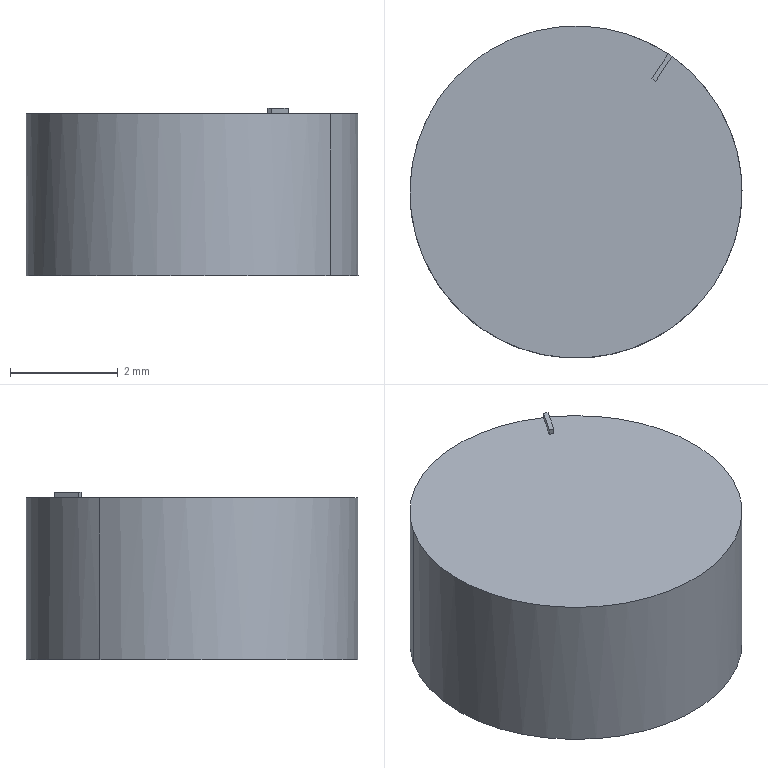Component | SolidWorks | Button-1 | 1 solid | 12 faces | box 6.16 x 6.16 x 3.1 mm | volume 88 mm3 | plane 8 | cylinder 4 | commonest cylinder face diameters 1 x2 6.16 x2
build123d program:
from build123d import *

# Parameters (mm, degrees)
SKETCH1_R           = 3.08
BOSS_EXTRUDE1_DEPTH = 3
SKETCH2_R           = 0.5
CUT_EXTRUDE1_DEPTH  = 2
SKETCH3_W           = 0.08765
SKETCH3_H           = 0.5469
BOSS_EXTRUDE2_DEPTH = 0.1


with BuildPart() as part:
    # Sketch1 → Boss-Extrude1 (new body)
    with BuildSketch(Plane.XY):
        Circle(SKETCH1_R)
    extrude(amount=BOSS_EXTRUDE1_DEPTH)

    # Sketch2 → Cut-Extrude1 (cut)
    with BuildSketch(Plane(origin=(0, 0, 0), x_dir=(-1, 0, 0), z_dir=(0, 0, -1))):
        Circle(SKETCH2_R)
    extrude(amount=-CUT_EXTRUDE1_DEPTH, mode=Mode.SUBTRACT)

    # Sketch3 → Boss-Extrude2 (add)
    with BuildSketch(Plane.XY.offset(3)):
        with Locations((0.04383, 2.807)):
            Rectangle(SKETCH3_W, SKETCH3_H)
    extrude(amount=BOSS_EXTRUDE2_DEPTH)


solid = part.part

# Placed as in the assembly
solid = solid.moved(Location((-92.68, 2.928, 277.152), (0.0002446, -0.0002387, -33.708)))
STEP:
#1=COLOUR_RGB('',0.7922,0.8196,0.9333);
#2=FILL_AREA_STYLE_COLOUR('',#1);
#3=FILL_AREA_STYLE('',(#2));
#4=SURFACE_STYLE_FILL_AREA(#3);
#5=SURFACE_SIDE_STYLE('',(#4));
#6=SURFACE_STYLE_USAGE(.BOTH.,#5);
#7=PRESENTATION_STYLE_ASSIGNMENT((#6));
#8=CARTESIAN_POINT('',(-3.632,0.1044,10.99));
#9=VERTEX_POINT('',#8);
#10=CARTESIAN_POINT('',(-3.665,0.1262,10.99));
#11=VERTEX_POINT('',#10);
#12=CARTESIAN_POINT('',(-3.649,0.1153,10.99));
#13=DIRECTION('',(0.,0.,-1.));
#14=DIRECTION('',(-0.8318,0.5551,0.));
#15=AXIS2_PLACEMENT_3D('',#12,#13,#14);
#16=CIRCLE('',#15,0.01969);
#17=EDGE_CURVE('',#9,#11,#16,.T.);
#18=ORIENTED_EDGE('',*,*,#17,.F.);
#19=CARTESIAN_POINT('',(-3.632,0.1044,10.911));
#20=VERTEX_POINT('',#19);
#21=CARTESIAN_POINT('',(-3.632,0.1044,10.99));
#22=DIRECTION('',(0.,0.,-1.));
#23=VECTOR('',#22,39.37);
#24=LINE('',#21,#23);
#25=EDGE_CURVE('',#9,#20,#24,.T.);
#26=ORIENTED_EDGE('',*,*,#25,.T.);
#27=CARTESIAN_POINT('',(-3.665,0.1262,10.911));
#28=VERTEX_POINT('',#27);
#29=CARTESIAN_POINT('',(-3.649,0.1153,10.911));
#30=DIRECTION('',(0.,0.,-1.));
#31=DIRECTION('',(-0.8318,0.5551,0.));
#32=AXIS2_PLACEMENT_3D('',#29,#30,#31);
#33=CIRCLE('',#32,0.01969);
#34=EDGE_CURVE('',#20,#28,#33,.T.);
#35=ORIENTED_EDGE('',*,*,#34,.T.);
#36=CARTESIAN_POINT('',(-3.665,0.1262,10.99));
#37=DIRECTION('',(0.,0.,-1.));
#38=VECTOR('',#37,39.37);
#39=LINE('',#36,#38);
#40=EDGE_CURVE('',#11,#28,#39,.T.);
#41=ORIENTED_EDGE('',*,*,#40,.F.);
#42=EDGE_LOOP('',(#18,#26,#35,#41));
#43=FACE_OUTER_BOUND('',#42,.T.);
#44=CARTESIAN_POINT('',(-3.649,0.1153,10.99));
#45=DIRECTION('',(0.,0.,-1.));
#46=DIRECTION('',(-0.8318,0.5551,0.));
#47=AXIS2_PLACEMENT_3D('',#44,#45,#46);
#48=CYLINDRICAL_SURFACE('',#47,0.01969);
#49=ADVANCED_FACE('',(#43),#48,.F.);
#50=CARTESIAN_POINT('',(-3.548,0.04799,11.03));
#51=VERTEX_POINT('',#50);
#52=CARTESIAN_POINT('',(-3.579,0.2142,11.03));
#53=VERTEX_POINT('',#52);
#54=CARTESIAN_POINT('',(-3.548,0.04799,11.03));
#55=CARTESIAN_POINT('',(-3.539,0.06111,11.03));
#56=CARTESIAN_POINT('',(-3.533,0.07541,11.03));
#57=CARTESIAN_POINT('',(-3.527,0.1063,11.03));
#58=CARTESIAN_POINT('',(-3.527,0.1218,11.03));
#59=CARTESIAN_POINT('',(-3.532,0.1528,11.03));
#60=CARTESIAN_POINT('',(-3.538,0.1673,11.03));
#61=CARTESIAN_POINT('',(-3.555,0.1938,11.03));
#62=CARTESIAN_POINT('',(-3.566,0.2051,11.03));
#63=CARTESIAN_POINT('',(-3.579,0.2142,11.03));
#64=B_SPLINE_CURVE_WITH_KNOTS('',3,(#54,#55,#56,#57,#58,#59,#60,#61,#62,#63),.UNSPECIFIED.,.F.,.F.,(4,2,2,2,4),(0.,0.06138,0.1228,0.1841,0.2455),.UNSPECIFIED.);
#65=EDGE_CURVE('',#51,#53,#64,.T.);
#66=ORIENTED_EDGE('',*,*,#65,.F.);
#67=CARTESIAN_POINT('',(-3.548,0.04799,10.911));
#68=VERTEX_POINT('',#67);
#69=CARTESIAN_POINT('',(-3.548,0.04799,11.03));
#70=DIRECTION('',(0.,0.,-1.));
#71=VECTOR('',#70,39.37);
#72=LINE('',#69,#71);
#73=EDGE_CURVE('',#51,#68,#72,.T.);
#74=ORIENTED_EDGE('',*,*,#73,.T.);
#75=CARTESIAN_POINT('',(-3.75,0.1826,10.911));
#76=VERTEX_POINT('',#75);
#77=CARTESIAN_POINT('',(-3.649,0.1153,10.911));
#78=DIRECTION('',(0.,0.,1.));
#79=DIRECTION('',(0.8318,-0.5551,0.));
#80=AXIS2_PLACEMENT_3D('',#77,#78,#79);
#81=CIRCLE('',#80,0.1213);
#82=EDGE_CURVE('',#68,#76,#81,.T.);
#83=ORIENTED_EDGE('',*,*,#82,.T.);
#84=CARTESIAN_POINT('',(-3.75,0.1826,11.03));
#85=VERTEX_POINT('',#84);
#86=CARTESIAN_POINT('',(-3.75,0.1826,11.03));
#87=DIRECTION('',(0.,0.,-1.));
#88=VECTOR('',#87,39.37);
#89=LINE('',#86,#88);
#90=EDGE_CURVE('',#85,#76,#89,.T.);
#91=ORIENTED_EDGE('',*,*,#90,.F.);
#92=CARTESIAN_POINT('',(-3.582,0.2162,11.03));
#93=VERTEX_POINT('',#92);
#94=CARTESIAN_POINT('',(-3.582,0.2162,11.03));
#95=CARTESIAN_POINT('',(-3.595,0.2251,11.03));
#96=CARTESIAN_POINT('',(-3.609,0.2311,11.03));
#97=CARTESIAN_POINT('',(-3.641,0.2374,11.03));
#98=CARTESIAN_POINT('',(-3.657,0.2373,11.03));
#99=CARTESIAN_POINT('',(-3.688,0.2311,11.03));
#100=CARTESIAN_POINT('',(-3.703,0.225,11.03));
#101=CARTESIAN_POINT('',(-3.73,0.2071,11.03));
#102=CARTESIAN_POINT('',(-3.741,0.196,11.03));
#103=CARTESIAN_POINT('',(-3.75,0.1826,11.03));
#104=B_SPLINE_CURVE_WITH_KNOTS('',3,(#94,#95,#96,#97,#98,#99,#100,#101,#102,#103),.UNSPECIFIED.,.F.,.F.,(4,2,2,2,4),(0.25,0.3125,0.375,0.4375,0.5),.UNSPECIFIED.);
#105=EDGE_CURVE('',#93,#85,#104,.T.);
#106=ORIENTED_EDGE('',*,*,#105,.F.);
#107=CARTESIAN_POINT('',(-3.579,0.2142,11.03));
#108=CARTESIAN_POINT('',(-3.58,0.2149,11.03));
#109=CARTESIAN_POINT('',(-3.581,0.2155,11.03));
#110=CARTESIAN_POINT('',(-3.582,0.2162,11.03));
#111=B_SPLINE_CURVE_WITH_KNOTS('',3,(#107,#108,#109,#110),.UNSPECIFIED.,.F.,.F.,(4,4),(0.,1.),.UNSPECIFIED.);
#112=EDGE_CURVE('',#53,#93,#111,.T.);
#113=ORIENTED_EDGE('',*,*,#112,.F.);
#114=EDGE_LOOP('',(#66,#74,#83,#91,#106,#113));
#115=FACE_OUTER_BOUND('',#114,.T.);
#116=CARTESIAN_POINT('',(-3.649,0.1153,11.03));
#117=DIRECTION('',(0.,0.,-1.));
#118=DIRECTION('',(-0.8318,0.5551,0.));
#119=AXIS2_PLACEMENT_3D('',#116,#117,#118);
#120=CYLINDRICAL_SURFACE('',#119,0.1213);
#121=ADVANCED_FACE('',(#115),#120,.T.);
#122=ORIENTED_EDGE('',*,*,#73,.F.);
#123=CARTESIAN_POINT('',(-3.75,0.1826,11.03));
#124=CARTESIAN_POINT('',(-3.759,0.1692,11.03));
#125=CARTESIAN_POINT('',(-3.765,0.1546,11.03));
#126=CARTESIAN_POINT('',(-3.771,0.1231,11.03));
#127=CARTESIAN_POINT('',(-3.771,0.1073,11.03));
#128=CARTESIAN_POINT('',(-3.765,0.07581,11.03));
#129=CARTESIAN_POINT('',(-3.759,0.06121,11.03));
#130=CARTESIAN_POINT('',(-3.741,0.03451,11.03));
#131=CARTESIAN_POINT('',(-3.729,0.02334,11.03));
#132=CARTESIAN_POINT('',(-3.703,0.005509,11.03));
#133=CARTESIAN_POINT('',(-3.688,-0.0005247,11.03));
#134=CARTESIAN_POINT('',(-3.657,-0.006779,11.03));
#135=CARTESIAN_POINT('',(-3.641,-0.006762,11.03));
#136=CARTESIAN_POINT('',(-3.609,-0.0004839,11.03));
#137=CARTESIAN_POINT('',(-3.595,0.005577,11.03));
#138=CARTESIAN_POINT('',(-3.568,0.02344,11.03));
#139=CARTESIAN_POINT('',(-3.557,0.0346,11.03));
#140=CARTESIAN_POINT('',(-3.548,0.04799,11.03));
#141=B_SPLINE_CURVE_WITH_KNOTS('',3,(#123,#124,#125,#126,#127,#128,#129,#130,#131,#132,#133,#134,#135,#136,#137,#138,#139,#140),.UNSPECIFIED.,.F.,.F.,(4,2,2,2,2,2,2,2,4),(0.5,0.5625,0.625,0.6875,0.75,0.8125,0.875,0.9375,1.),.UNSPECIFIED.);
#142=EDGE_CURVE('',#85,#51,#141,.T.);
#143=ORIENTED_EDGE('',*,*,#142,.F.);
#144=ORIENTED_EDGE('',*,*,#90,.T.);
#145=CARTESIAN_POINT('',(-3.649,0.1153,10.911));
#146=DIRECTION('',(0.,0.,1.));
#147=DIRECTION('',(0.8318,-0.5551,0.));
#148=AXIS2_PLACEMENT_3D('',#145,#146,#147);
#149=CIRCLE('',#148,0.1213);
#150=EDGE_CURVE('',#76,#68,#149,.T.);
#151=ORIENTED_EDGE('',*,*,#150,.T.);
#152=EDGE_LOOP('',(#122,#143,#144,#151));
#153=FACE_OUTER_BOUND('',#152,.T.);
#154=CARTESIAN_POINT('',(-3.649,0.1153,11.03));
#155=DIRECTION('',(0.,0.,-1.));
#156=DIRECTION('',(-0.8318,0.5551,0.));
#157=AXIS2_PLACEMENT_3D('',#154,#155,#156);
#158=CYLINDRICAL_SURFACE('',#157,0.1213);
#159=ADVANCED_FACE('',(#153),#158,.T.);
#160=CARTESIAN_POINT('',(-3.593,0.1982,11.03));
#161=VERTEX_POINT('',#160);
#162=CARTESIAN_POINT('',(-3.582,0.2162,11.03));
#163=DIRECTION('',(-0.5551,-0.8318,0.));
#164=VECTOR('',#163,39.37);
#165=LINE('',#162,#164);
#166=EDGE_CURVE('',#93,#161,#165,.T.);
#167=ORIENTED_EDGE('',*,*,#166,.F.);
#168=ORIENTED_EDGE('',*,*,#105,.T.);
#169=ORIENTED_EDGE('',*,*,#142,.T.);
#170=ORIENTED_EDGE('',*,*,#65,.T.);
#171=CARTESIAN_POINT('',(-3.591,0.1963,11.03));
#172=VERTEX_POINT('',#171);
#173=CARTESIAN_POINT('',(-3.579,0.2142,11.03));
#174=DIRECTION('',(0.5551,0.8318,0.));
#175=VECTOR('',#174,39.37);
#176=LINE('',#173,#175);
#177=EDGE_CURVE('',#172,#53,#176,.T.);
#178=ORIENTED_EDGE('',*,*,#177,.F.);
#179=CARTESIAN_POINT('',(-3.593,0.1982,11.03));
#180=DIRECTION('',(0.8318,-0.5551,0.));
#181=VECTOR('',#180,39.37);
#182=LINE('',#179,#181);
#183=EDGE_CURVE('',#161,#172,#182,.T.);
#184=ORIENTED_EDGE('',*,*,#183,.F.);
#185=EDGE_LOOP('',(#167,#168,#169,#170,#178,#184));
#186=FACE_OUTER_BOUND('',#185,.T.);
#187=CARTESIAN_POINT('',(-3.649,0.1153,11.03));
#188=DIRECTION('',(0.,0.,1.));
#189=DIRECTION('',(0.8318,-0.5551,0.));
#190=AXIS2_PLACEMENT_3D('',#187,#188,#189);
#191=PLANE('',#190);
#192=ADVANCED_FACE('',(#186),#191,.T.);
#193=CARTESIAN_POINT('',(-3.649,0.1153,10.911));
#194=DIRECTION('',(0.,0.,-1.));
#195=DIRECTION('',(-0.8318,0.5551,0.));
#196=AXIS2_PLACEMENT_3D('',#193,#194,#195);
#197=CIRCLE('',#196,0.01969);
#198=EDGE_CURVE('',#28,#20,#197,.T.);
#199=ORIENTED_EDGE('',*,*,#198,.F.);
#200=ORIENTED_EDGE('',*,*,#34,.F.);
#201=EDGE_LOOP('',(#199,#200));
#202=FACE_BOUND('',#201,.T.);
#203=ORIENTED_EDGE('',*,*,#150,.F.);
#204=ORIENTED_EDGE('',*,*,#82,.F.);
#205=EDGE_LOOP('',(#203,#204));
#206=FACE_OUTER_BOUND('',#205,.T.);
#207=CARTESIAN_POINT('',(-3.649,0.1153,10.911));
#208=DIRECTION('',(0.,0.,1.));
#209=DIRECTION('',(0.8318,-0.5551,0.));
#210=AXIS2_PLACEMENT_3D('',#207,#208,#209);
#211=PLANE('',#210);
#212=ADVANCED_FACE('',(#202,#206),#211,.F.);
#213=ORIENTED_EDGE('',*,*,#25,.F.);
#214=CARTESIAN_POINT('',(-3.649,0.1153,10.99));
#215=DIRECTION('',(0.,0.,-1.));
#216=DIRECTION('',(-0.8318,0.5551,0.));
#217=AXIS2_PLACEMENT_3D('',#214,#215,#216);
#218=CIRCLE('',#217,0.01969);
#219=EDGE_CURVE('',#11,#9,#218,.T.);
#220=ORIENTED_EDGE('',*,*,#219,.F.);
#221=ORIENTED_EDGE('',*,*,#40,.T.);
#222=ORIENTED_EDGE('',*,*,#198,.T.);
#223=EDGE_LOOP('',(#213,#220,#221,#222));
#224=FACE_OUTER_BOUND('',#223,.T.);
#225=CARTESIAN_POINT('',(-3.649,0.1153,10.99));
#226=DIRECTION('',(0.,0.,-1.));
#227=DIRECTION('',(-0.8318,0.5551,0.));
#228=AXIS2_PLACEMENT_3D('',#225,#226,#227);
#229=CYLINDRICAL_SURFACE('',#228,0.01969);
#230=ADVANCED_FACE('',(#224),#229,.F.);
#231=ORIENTED_EDGE('',*,*,#219,.T.);
#232=ORIENTED_EDGE('',*,*,#17,.T.);
#233=EDGE_LOOP('',(#231,#232));
#234=FACE_OUTER_BOUND('',#233,.T.);
#235=CARTESIAN_POINT('',(-3.649,0.1153,10.99));
#236=DIRECTION('',(0.,0.,-1.));
#237=DIRECTION('',(-0.8318,0.5551,0.));
#238=AXIS2_PLACEMENT_3D('',#235,#236,#237);
#239=PLANE('',#238);
#240=ADVANCED_FACE('',(#234),#239,.T.);
#241=ORIENTED_EDGE('',*,*,#166,.T.);
#242=CARTESIAN_POINT('',(-3.593,0.1982,11.034));
#243=VERTEX_POINT('',#242);
#244=CARTESIAN_POINT('',(-3.593,0.1982,11.034));
#245=DIRECTION('',(0.,0.,-1.));
#246=VECTOR('',#245,39.37);
#247=LINE('',#244,#246);
#248=EDGE_CURVE('',#243,#161,#247,.T.);
#249=ORIENTED_EDGE('',*,*,#248,.F.);
#250=CARTESIAN_POINT('',(-3.582,0.2162,11.034));
#251=VERTEX_POINT('',#250);
#252=CARTESIAN_POINT('',(-3.582,0.2162,11.034));
#253=DIRECTION('',(-0.5551,-0.8318,0.));
#254=VECTOR('',#253,39.37);
#255=LINE('',#252,#254);
#256=EDGE_CURVE('',#251,#243,#255,.T.);
#257=ORIENTED_EDGE('',*,*,#256,.F.);
#258=CARTESIAN_POINT('',(-3.582,0.2162,11.034));
#259=DIRECTION('',(0.,0.,-1.));
#260=VECTOR('',#259,39.37);
#261=LINE('',#258,#260);
#262=EDGE_CURVE('',#251,#93,#261,.T.);
#263=ORIENTED_EDGE('',*,*,#262,.T.);
#264=EDGE_LOOP('',(#241,#249,#257,#263));
#265=FACE_OUTER_BOUND('',#264,.T.);
#266=CARTESIAN_POINT('',(-3.582,0.2162,11.034));
#267=DIRECTION('',(0.8318,-0.5551,0.));
#268=DIRECTION('',(0.,0.,-1.));
#269=AXIS2_PLACEMENT_3D('',#266,#267,#268);
#270=PLANE('',#269);
#271=ADVANCED_FACE('',(#265),#270,.F.);
#272=ORIENTED_EDGE('',*,*,#183,.T.);
#273=CARTESIAN_POINT('',(-3.591,0.1963,11.034));
#274=VERTEX_POINT('',#273);
#275=CARTESIAN_POINT('',(-3.591,0.1963,11.034));
#276=DIRECTION('',(0.,0.,-1.));
#277=VECTOR('',#276,39.37);
#278=LINE('',#275,#277);
#279=EDGE_CURVE('',#274,#172,#278,.T.);
#280=ORIENTED_EDGE('',*,*,#279,.F.);
#281=CARTESIAN_POINT('',(-3.593,0.1982,11.034));
#282=DIRECTION('',(0.8318,-0.5551,0.));
#283=VECTOR('',#282,39.37);
#284=LINE('',#281,#283);
#285=EDGE_CURVE('',#243,#274,#284,.T.);
#286=ORIENTED_EDGE('',*,*,#285,.F.);
#287=ORIENTED_EDGE('',*,*,#248,.T.);
#288=EDGE_LOOP('',(#272,#280,#286,#287));
#289=FACE_OUTER_BOUND('',#288,.T.);
#290=CARTESIAN_POINT('',(-3.593,0.1982,11.034));
#291=DIRECTION('',(0.5551,0.8318,0.));
#292=DIRECTION('',(0.,0.,1.));
#293=AXIS2_PLACEMENT_3D('',#290,#291,#292);
#294=PLANE('',#293);
#295=ADVANCED_FACE('',(#289),#294,.F.);
#296=ORIENTED_EDGE('',*,*,#177,.T.);
#297=CARTESIAN_POINT('',(-3.579,0.2142,11.034));
#298=VERTEX_POINT('',#297);
#299=CARTESIAN_POINT('',(-3.579,0.2142,11.034));
#300=DIRECTION('',(0.,0.,-1.));
#301=VECTOR('',#300,39.37);
#302=LINE('',#299,#301);
#303=EDGE_CURVE('',#298,#53,#302,.T.);
#304=ORIENTED_EDGE('',*,*,#303,.F.);
#305=CARTESIAN_POINT('',(-3.579,0.2142,11.034));
#306=DIRECTION('',(0.5551,0.8318,0.));
#307=VECTOR('',#306,39.37);
#308=LINE('',#305,#307);
#309=EDGE_CURVE('',#274,#298,#308,.T.);
#310=ORIENTED_EDGE('',*,*,#309,.F.);
#311=ORIENTED_EDGE('',*,*,#279,.T.);
#312=EDGE_LOOP('',(#296,#304,#310,#311));
#313=FACE_OUTER_BOUND('',#312,.T.);
#314=CARTESIAN_POINT('',(-3.579,0.2142,11.034));
#315=DIRECTION('',(-0.8318,0.5551,0.));
#316=DIRECTION('',(0.,0.,1.));
#317=AXIS2_PLACEMENT_3D('',#314,#315,#316);
#318=PLANE('',#317);
#319=ADVANCED_FACE('',(#313),#318,.F.);
#320=ORIENTED_EDGE('',*,*,#112,.T.);
#321=ORIENTED_EDGE('',*,*,#262,.F.);
#322=CARTESIAN_POINT('',(-3.582,0.2162,11.034));
#323=DIRECTION('',(-0.8318,0.5551,0.));
#324=VECTOR('',#323,39.37);
#325=LINE('',#322,#324);
#326=EDGE_CURVE('',#298,#251,#325,.T.);
#327=ORIENTED_EDGE('',*,*,#326,.F.);
#328=ORIENTED_EDGE('',*,*,#303,.T.);
#329=EDGE_LOOP('',(#320,#321,#327,#328));
#330=FACE_OUTER_BOUND('',#329,.T.);
#331=CARTESIAN_POINT('',(-3.582,0.2162,11.034));
#332=DIRECTION('',(-0.5551,-0.8318,0.));
#333=DIRECTION('',(0.,0.,-1.));
#334=AXIS2_PLACEMENT_3D('',#331,#332,#333);
#335=PLANE('',#334);
#336=ADVANCED_FACE('',(#330),#335,.F.);
#337=ORIENTED_EDGE('',*,*,#256,.T.);
#338=ORIENTED_EDGE('',*,*,#285,.T.);
#339=ORIENTED_EDGE('',*,*,#309,.T.);
#340=ORIENTED_EDGE('',*,*,#326,.T.);
#341=EDGE_LOOP('',(#337,#338,#339,#340));
#342=FACE_OUTER_BOUND('',#341,.T.);
#343=CARTESIAN_POINT('',(-3.649,0.1153,11.034));
#344=DIRECTION('',(0.,0.,1.));
#345=DIRECTION('',(0.8318,-0.5551,0.));
#346=AXIS2_PLACEMENT_3D('',#343,#344,#345);
#347=PLANE('',#346);
#348=ADVANCED_FACE('',(#342),#347,.T.);
#349=CLOSED_SHELL('',(#49,#121,#159,#192,#212,#230,#240,#271,#295,#319,#336,#348));
#350=MANIFOLD_SOLID_BREP('',#349);
#351=STYLED_ITEM('',(#7),#350);
#352=(LENGTH_UNIT()NAMED_UNIT(*)SI_UNIT($,.METRE.));
#353=LENGTH_MEASURE_WITH_UNIT(LENGTH_MEASURE(0.0254),#352);
#354=DIMENSIONAL_EXPONENTS(1.,0.,0.,0.,0.,0.,0.);
#355=(CONVERSION_BASED_UNIT('',#353)LENGTH_UNIT()NAMED_UNIT(#354));
#356=UNCERTAINTY_MEASURE_WITH_UNIT(LENGTH_MEASURE(0.00001),#355,'','');
#357=(NAMED_UNIT(*)PLANE_ANGLE_UNIT()SI_UNIT($,.RADIAN.));
#358=(NAMED_UNIT(*)SI_UNIT($,.STERADIAN.)SOLID_ANGLE_UNIT());
#359=(GEOMETRIC_REPRESENTATION_CONTEXT(3)GLOBAL_UNCERTAINTY_ASSIGNED_CONTEXT((#356))GLOBAL_UNIT_ASSIGNED_CONTEXT((#355,#357,#358))REPRESENTATION_CONTEXT('',''));
#360=MECHANICAL_DESIGN_GEOMETRIC_PRESENTATION_REPRESENTATION('',(#351),#359);
#361=CARTESIAN_POINT('',(0.,0.,0.));
#362=DIRECTION('',(0.,0.,1.));
#363=DIRECTION('',(1.,0.,0.));
#364=AXIS2_PLACEMENT_3D('',#361,#362,#363);
#365=(LENGTH_UNIT()NAMED_UNIT(*)SI_UNIT($,.METRE.));
#366=LENGTH_MEASURE_WITH_UNIT(LENGTH_MEASURE(0.0254),#365);
#367=DIMENSIONAL_EXPONENTS(1.,0.,0.,0.,0.,0.,0.);
#368=(CONVERSION_BASED_UNIT('',#366)LENGTH_UNIT()NAMED_UNIT(#367));
#369=UNCERTAINTY_MEASURE_WITH_UNIT(LENGTH_MEASURE(0.00001),#368,'','');
#370=(NAMED_UNIT(*)PLANE_ANGLE_UNIT()SI_UNIT($,.RADIAN.));
#371=(NAMED_UNIT(*)SI_UNIT($,.STERADIAN.)SOLID_ANGLE_UNIT());
#372=(GEOMETRIC_REPRESENTATION_CONTEXT(3)GLOBAL_UNCERTAINTY_ASSIGNED_CONTEXT((#369))GLOBAL_UNIT_ASSIGNED_CONTEXT((#368,#370,#371))REPRESENTATION_CONTEXT('',''));
#373=ADVANCED_BREP_SHAPE_REPRESENTATION('',(#350,#364),#372);
#374=PRESENTATION_LAYER_ASSIGNMENT('','',(#351));